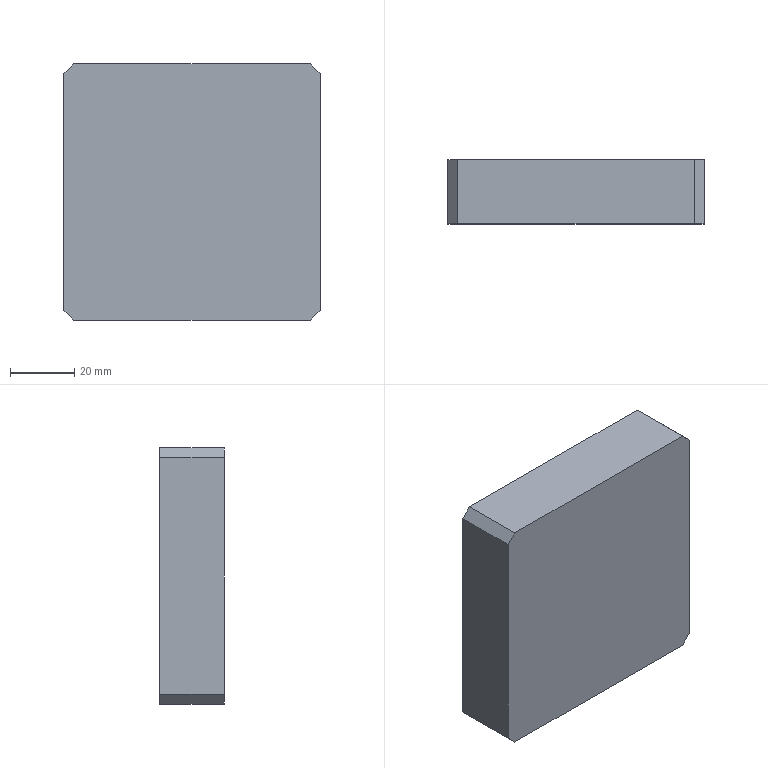Component | SolidWorks | CoilCarrier-10 | 1 solid | 24 faces | box 80 x 20 x 80 mm | volume 111580 mm3 | plane 24 | material Plain Carbon Steel
build123d program:
from build123d import *

# Parameters (mm, degrees)
SKETCH1_W           = 80
SKETCH1_H           = 80
BOSS_EXTRUDE1_DEPTH = 20
CUT_EXTRUDE1_DEPTH  = 11
CHAMFER1_SIZE       = 3
SKETCH3_W           = 14
SKETCH3_H           = 22
CUT_EXTRUDE2_DEPTH  = 1.25


with BuildPart() as part:
    # Sketch1 → Boss-Extrude1 (new body)
    with BuildSketch(Plane.XY):
        Rectangle(SKETCH1_W, SKETCH1_H)
    extrude(amount=BOSS_EXTRUDE1_DEPTH)

    # Sketch2 → Cut-Extrude1 (cut)
    with BuildSketch(Plane.XY.offset(20)):
        Polygon((12.5, -6), (12.5, -18), (-19.5, -18), (-19.5, -23), (-27.5, -23), (-27.5, -18), (-32.5, -18), (-32.5, -6), (-20, -6), (-20, 20), (-10.75, 20), (3.25, 20), (12.5, 20), align=None)
    extrude(amount=-CUT_EXTRUDE1_DEPTH, mode=Mode.SUBTRACT)

    # Chamfer1
    chamfer1_edges = [part.edges().sort_by_distance(p)[0] for p in [
        (-40, 40, 10),
        (40, 40, 10),
        (40, -40, 10),
        (-40, -40, 10),
    ]]
    chamfer(chamfer1_edges, length=CHAMFER1_SIZE)

    # Sketch3 → Cut-Extrude2 (cut)
    with BuildSketch(Plane.XY.offset(20)):
        with Locations((-3.75, -29)):
            Rectangle(SKETCH3_W, SKETCH3_H)
    extrude(amount=-CUT_EXTRUDE2_DEPTH, mode=Mode.SUBTRACT)


solid = part.part

# Placed as in the assembly
solid = solid.moved(Location((-4.55, 27.146, 668.775), (-90, 0, 90)))
STEP:
#1=COLOUR_RGB('',0.7922,0.8196,0.9333);
#2=FILL_AREA_STYLE_COLOUR('',#1);
#3=FILL_AREA_STYLE('',(#2));
#4=SURFACE_STYLE_FILL_AREA(#3);
#5=SURFACE_SIDE_STYLE('',(#4));
#6=SURFACE_STYLE_USAGE(.BOTH.,#5);
#7=PRESENTATION_STYLE_ASSIGNMENT((#6));
#8=CARTESIAN_POINT('',(-1.636,1.856,27.905));
#9=VERTEX_POINT('',#8);
#10=CARTESIAN_POINT('',(1.278,1.856,27.905));
#11=VERTEX_POINT('',#10);
#12=CARTESIAN_POINT('',(1.396,1.856,27.905));
#13=DIRECTION('',(1.,0.,0.));
#14=VECTOR('',#13,39.37);
#15=LINE('',#12,#14);
#16=EDGE_CURVE('',#9,#11,#15,.T.);
#17=ORIENTED_EDGE('',*,*,#16,.F.);
#18=CARTESIAN_POINT('',(-1.636,1.069,27.905));
#19=VERTEX_POINT('',#18);
#20=CARTESIAN_POINT('',(-1.636,1.856,27.905));
#21=DIRECTION('',(0.,-1.,-0.));
#22=VECTOR('',#21,39.37);
#23=LINE('',#20,#22);
#24=EDGE_CURVE('',#9,#19,#23,.T.);
#25=ORIENTED_EDGE('',*,*,#24,.T.);
#26=CARTESIAN_POINT('',(1.278,1.069,27.905));
#27=VERTEX_POINT('',#26);
#28=CARTESIAN_POINT('',(1.396,1.069,27.905));
#29=DIRECTION('',(1.,0.,0.));
#30=VECTOR('',#29,39.37);
#31=LINE('',#28,#30);
#32=EDGE_CURVE('',#19,#27,#31,.T.);
#33=ORIENTED_EDGE('',*,*,#32,.T.);
#34=CARTESIAN_POINT('',(1.278,1.856,27.905));
#35=DIRECTION('',(-0.,1.,0.));
#36=VECTOR('',#35,39.37);
#37=LINE('',#34,#36);
#38=EDGE_CURVE('',#27,#11,#37,.T.);
#39=ORIENTED_EDGE('',*,*,#38,.T.);
#40=EDGE_LOOP('',(#17,#25,#33,#39));
#41=FACE_OUTER_BOUND('',#40,.T.);
#42=CARTESIAN_POINT('',(1.396,1.856,27.905));
#43=DIRECTION('',(0.,0.,-1.));
#44=DIRECTION('',(0.,-1.,-0.));
#45=AXIS2_PLACEMENT_3D('',#42,#43,#44);
#46=PLANE('',#45);
#47=ADVANCED_FACE('',(#41),#46,.F.);
#48=CARTESIAN_POINT('',(1.396,1.807,26.753));
#49=VERTEX_POINT('',#48);
#50=CARTESIAN_POINT('',(1.396,1.807,26.202));
#51=VERTEX_POINT('',#50);
#52=CARTESIAN_POINT('',(1.396,1.807,26.753));
#53=DIRECTION('',(0.,0.,-1.));
#54=VECTOR('',#53,39.37);
#55=LINE('',#52,#54);
#56=EDGE_CURVE('',#49,#51,#55,.T.);
#57=ORIENTED_EDGE('',*,*,#56,.F.);
#58=CARTESIAN_POINT('',(1.396,1.856,26.753));
#59=VERTEX_POINT('',#58);
#60=CARTESIAN_POINT('',(1.396,1.807,26.753));
#61=DIRECTION('',(-0.,1.,0.));
#62=VECTOR('',#61,39.37);
#63=LINE('',#60,#62);
#64=EDGE_CURVE('',#49,#59,#63,.T.);
#65=ORIENTED_EDGE('',*,*,#64,.T.);
#66=CARTESIAN_POINT('',(1.396,1.856,27.786));
#67=VERTEX_POINT('',#66);
#68=CARTESIAN_POINT('',(1.396,1.856,24.755));
#69=DIRECTION('',(0.,0.,-1.));
#70=VECTOR('',#69,39.37);
#71=LINE('',#68,#70);
#72=EDGE_CURVE('',#67,#59,#71,.T.);
#73=ORIENTED_EDGE('',*,*,#72,.F.);
#74=CARTESIAN_POINT('',(1.396,1.069,27.786));
#75=VERTEX_POINT('',#74);
#76=CARTESIAN_POINT('',(1.396,1.856,27.786));
#77=DIRECTION('',(0.,-1.,-0.));
#78=VECTOR('',#77,39.37);
#79=LINE('',#76,#78);
#80=EDGE_CURVE('',#67,#75,#79,.T.);
#81=ORIENTED_EDGE('',*,*,#80,.T.);
#82=CARTESIAN_POINT('',(1.396,1.069,24.873));
#83=VERTEX_POINT('',#82);
#84=CARTESIAN_POINT('',(1.396,1.069,24.755));
#85=DIRECTION('',(0.,0.,-1.));
#86=VECTOR('',#85,39.37);
#87=LINE('',#84,#86);
#88=EDGE_CURVE('',#75,#83,#87,.T.);
#89=ORIENTED_EDGE('',*,*,#88,.T.);
#90=CARTESIAN_POINT('',(1.396,1.856,24.873));
#91=VERTEX_POINT('',#90);
#92=CARTESIAN_POINT('',(1.396,1.856,24.873));
#93=DIRECTION('',(-0.,1.,0.));
#94=VECTOR('',#93,39.37);
#95=LINE('',#92,#94);
#96=EDGE_CURVE('',#83,#91,#95,.T.);
#97=ORIENTED_EDGE('',*,*,#96,.T.);
#98=CARTESIAN_POINT('',(1.396,1.856,26.202));
#99=VERTEX_POINT('',#98);
#100=CARTESIAN_POINT('',(1.396,1.856,24.755));
#101=DIRECTION('',(0.,0.,-1.));
#102=VECTOR('',#101,39.37);
#103=LINE('',#100,#102);
#104=EDGE_CURVE('',#99,#91,#103,.T.);
#105=ORIENTED_EDGE('',*,*,#104,.F.);
#106=CARTESIAN_POINT('',(1.396,1.807,26.202));
#107=DIRECTION('',(-0.,1.,0.));
#108=VECTOR('',#107,39.37);
#109=LINE('',#106,#108);
#110=EDGE_CURVE('',#51,#99,#109,.T.);
#111=ORIENTED_EDGE('',*,*,#110,.F.);
#112=EDGE_LOOP('',(#57,#65,#73,#81,#89,#97,#105,#111));
#113=FACE_OUTER_BOUND('',#112,.T.);
#114=CARTESIAN_POINT('',(1.396,1.856,24.755));
#115=DIRECTION('',(-1.,-0.,-0.));
#116=DIRECTION('',(-0.,-0.,1.));
#117=AXIS2_PLACEMENT_3D('',#114,#115,#116);
#118=PLANE('',#117);
#119=ADVANCED_FACE('',(#113),#118,.F.);
#120=CARTESIAN_POINT('',(1.278,1.069,24.755));
#121=VERTEX_POINT('',#120);
#122=CARTESIAN_POINT('',(-1.636,1.069,24.755));
#123=VERTEX_POINT('',#122);
#124=CARTESIAN_POINT('',(1.396,1.069,24.755));
#125=DIRECTION('',(-1.,-0.,-0.));
#126=VECTOR('',#125,39.37);
#127=LINE('',#124,#126);
#128=EDGE_CURVE('',#121,#123,#127,.T.);
#129=ORIENTED_EDGE('',*,*,#128,.T.);
#130=CARTESIAN_POINT('',(-1.636,1.856,24.755));
#131=VERTEX_POINT('',#130);
#132=CARTESIAN_POINT('',(-1.636,1.856,24.755));
#133=DIRECTION('',(-0.,1.,0.));
#134=VECTOR('',#133,39.37);
#135=LINE('',#132,#134);
#136=EDGE_CURVE('',#123,#131,#135,.T.);
#137=ORIENTED_EDGE('',*,*,#136,.T.);
#138=CARTESIAN_POINT('',(1.278,1.856,24.755));
#139=VERTEX_POINT('',#138);
#140=CARTESIAN_POINT('',(1.396,1.856,24.755));
#141=DIRECTION('',(-1.,-0.,-0.));
#142=VECTOR('',#141,39.37);
#143=LINE('',#140,#142);
#144=EDGE_CURVE('',#139,#131,#143,.T.);
#145=ORIENTED_EDGE('',*,*,#144,.F.);
#146=CARTESIAN_POINT('',(1.278,1.856,24.755));
#147=DIRECTION('',(0.,-1.,-0.));
#148=VECTOR('',#147,39.37);
#149=LINE('',#146,#148);
#150=EDGE_CURVE('',#139,#121,#149,.T.);
#151=ORIENTED_EDGE('',*,*,#150,.T.);
#152=EDGE_LOOP('',(#129,#137,#145,#151));
#153=FACE_OUTER_BOUND('',#152,.T.);
#154=CARTESIAN_POINT('',(1.396,1.856,24.755));
#155=DIRECTION('',(-0.,-0.,1.));
#156=DIRECTION('',(-0.,1.,0.));
#157=AXIS2_PLACEMENT_3D('',#154,#155,#156);
#158=PLANE('',#157);
#159=ADVANCED_FACE('',(#153),#158,.F.);
#160=CARTESIAN_POINT('',(-1.754,1.856,24.873));
#161=VERTEX_POINT('',#160);
#162=CARTESIAN_POINT('',(-1.754,1.856,27.786));
#163=VERTEX_POINT('',#162);
#164=CARTESIAN_POINT('',(-1.754,1.856,24.755));
#165=DIRECTION('',(0.,-0.,1.));
#166=VECTOR('',#165,39.37);
#167=LINE('',#164,#166);
#168=EDGE_CURVE('',#161,#163,#167,.T.);
#169=ORIENTED_EDGE('',*,*,#168,.F.);
#170=CARTESIAN_POINT('',(-1.754,1.069,24.873));
#171=VERTEX_POINT('',#170);
#172=CARTESIAN_POINT('',(-1.754,1.856,24.873));
#173=DIRECTION('',(0.,-1.,-0.));
#174=VECTOR('',#173,39.37);
#175=LINE('',#172,#174);
#176=EDGE_CURVE('',#161,#171,#175,.T.);
#177=ORIENTED_EDGE('',*,*,#176,.T.);
#178=CARTESIAN_POINT('',(-1.754,1.069,27.786));
#179=VERTEX_POINT('',#178);
#180=CARTESIAN_POINT('',(-1.754,1.069,24.755));
#181=DIRECTION('',(0.,-0.,1.));
#182=VECTOR('',#181,39.37);
#183=LINE('',#180,#182);
#184=EDGE_CURVE('',#171,#179,#183,.T.);
#185=ORIENTED_EDGE('',*,*,#184,.T.);
#186=CARTESIAN_POINT('',(-1.754,1.856,27.786));
#187=DIRECTION('',(-0.,1.,0.));
#188=VECTOR('',#187,39.37);
#189=LINE('',#186,#188);
#190=EDGE_CURVE('',#179,#163,#189,.T.);
#191=ORIENTED_EDGE('',*,*,#190,.T.);
#192=EDGE_LOOP('',(#169,#177,#185,#191));
#193=FACE_OUTER_BOUND('',#192,.T.);
#194=CARTESIAN_POINT('',(-1.754,1.856,24.755));
#195=DIRECTION('',(1.,0.,-0.));
#196=DIRECTION('',(-0.,0.,-1.));
#197=AXIS2_PLACEMENT_3D('',#194,#195,#196);
#198=PLANE('',#197);
#199=ADVANCED_FACE('',(#193),#198,.F.);
#200=CARTESIAN_POINT('',(0.5295,1.856,26.753));
#201=VERTEX_POINT('',#200);
#202=CARTESIAN_POINT('',(0.5295,1.856,26.753));
#203=DIRECTION('',(1.,0.,0.));
#204=VECTOR('',#203,39.37);
#205=LINE('',#202,#204);
#206=EDGE_CURVE('',#201,#59,#205,.T.);
#207=ORIENTED_EDGE('',*,*,#206,.F.);
#208=CARTESIAN_POINT('',(0.5295,1.856,27.097));
#209=VERTEX_POINT('',#208);
#210=CARTESIAN_POINT('',(0.5295,1.856,25.838));
#211=DIRECTION('',(0.,0.,-1.));
#212=VECTOR('',#211,39.37);
#213=LINE('',#210,#212);
#214=EDGE_CURVE('',#209,#201,#213,.T.);
#215=ORIENTED_EDGE('',*,*,#214,.F.);
#216=CARTESIAN_POINT('',(0.7264,1.856,27.097));
#217=VERTEX_POINT('',#216);
#218=CARTESIAN_POINT('',(0.5295,1.856,27.097));
#219=DIRECTION('',(-1.,-0.,-0.));
#220=VECTOR('',#219,39.37);
#221=LINE('',#218,#220);
#222=EDGE_CURVE('',#217,#209,#221,.T.);
#223=ORIENTED_EDGE('',*,*,#222,.F.);
#224=CARTESIAN_POINT('',(0.7264,1.856,27.412));
#225=VERTEX_POINT('',#224);
#226=CARTESIAN_POINT('',(0.7264,1.856,27.412));
#227=DIRECTION('',(0.,0.,-1.));
#228=VECTOR('',#227,39.37);
#229=LINE('',#226,#228);
#230=EDGE_CURVE('',#225,#217,#229,.T.);
#231=ORIENTED_EDGE('',*,*,#230,.F.);
#232=CARTESIAN_POINT('',(0.5295,1.856,27.412));
#233=VERTEX_POINT('',#232);
#234=CARTESIAN_POINT('',(0.5295,1.856,27.412));
#235=DIRECTION('',(1.,0.,0.));
#236=VECTOR('',#235,39.37);
#237=LINE('',#234,#236);
#238=EDGE_CURVE('',#233,#225,#237,.T.);
#239=ORIENTED_EDGE('',*,*,#238,.F.);
#240=CARTESIAN_POINT('',(0.5295,1.856,27.609));
#241=VERTEX_POINT('',#240);
#242=CARTESIAN_POINT('',(0.5295,1.856,27.609));
#243=DIRECTION('',(0.,0.,-1.));
#244=VECTOR('',#243,39.37);
#245=LINE('',#242,#244);
#246=EDGE_CURVE('',#241,#233,#245,.T.);
#247=ORIENTED_EDGE('',*,*,#246,.F.);
#248=CARTESIAN_POINT('',(0.0571,1.856,27.609));
#249=VERTEX_POINT('',#248);
#250=CARTESIAN_POINT('',(0.0571,1.856,27.609));
#251=DIRECTION('',(1.,0.,0.));
#252=VECTOR('',#251,39.37);
#253=LINE('',#250,#252);
#254=EDGE_CURVE('',#249,#241,#253,.T.);
#255=ORIENTED_EDGE('',*,*,#254,.F.);
#256=CARTESIAN_POINT('',(0.0571,1.856,27.117));
#257=VERTEX_POINT('',#256);
#258=CARTESIAN_POINT('',(0.0571,1.856,27.117));
#259=DIRECTION('',(-0.,-0.,1.));
#260=VECTOR('',#259,39.37);
#261=LINE('',#258,#260);
#262=EDGE_CURVE('',#257,#249,#261,.T.);
#263=ORIENTED_EDGE('',*,*,#262,.F.);
#264=CARTESIAN_POINT('',(-0.9665,1.856,27.117));
#265=VERTEX_POINT('',#264);
#266=CARTESIAN_POINT('',(0.0571,1.856,27.117));
#267=DIRECTION('',(1.,0.,0.));
#268=VECTOR('',#267,39.37);
#269=LINE('',#266,#268);
#270=EDGE_CURVE('',#265,#257,#269,.T.);
#271=ORIENTED_EDGE('',*,*,#270,.F.);
#272=CARTESIAN_POINT('',(-0.9665,1.856,25.838));
#273=VERTEX_POINT('',#272);
#274=CARTESIAN_POINT('',(-0.9665,1.856,26.753));
#275=DIRECTION('',(-0.,-0.,1.));
#276=VECTOR('',#275,39.37);
#277=LINE('',#274,#276);
#278=EDGE_CURVE('',#273,#265,#277,.T.);
#279=ORIENTED_EDGE('',*,*,#278,.F.);
#280=CARTESIAN_POINT('',(0.5295,1.856,25.838));
#281=VERTEX_POINT('',#280);
#282=CARTESIAN_POINT('',(0.0571,1.856,25.838));
#283=DIRECTION('',(-1.,-0.,-0.));
#284=VECTOR('',#283,39.37);
#285=LINE('',#282,#284);
#286=EDGE_CURVE('',#281,#273,#285,.T.);
#287=ORIENTED_EDGE('',*,*,#286,.F.);
#288=CARTESIAN_POINT('',(0.5295,1.856,26.202));
#289=VERTEX_POINT('',#288);
#290=CARTESIAN_POINT('',(0.5295,1.856,25.838));
#291=DIRECTION('',(0.,0.,-1.));
#292=VECTOR('',#291,39.37);
#293=LINE('',#290,#292);
#294=EDGE_CURVE('',#289,#281,#293,.T.);
#295=ORIENTED_EDGE('',*,*,#294,.F.);
#296=CARTESIAN_POINT('',(0.5295,1.856,26.202));
#297=DIRECTION('',(-1.,-0.,0.));
#298=VECTOR('',#297,39.37);
#299=LINE('',#296,#298);
#300=EDGE_CURVE('',#99,#289,#299,.T.);
#301=ORIENTED_EDGE('',*,*,#300,.F.);
#302=ORIENTED_EDGE('',*,*,#104,.T.);
#303=CARTESIAN_POINT('',(1.337,1.856,24.814));
#304=DIRECTION('',(-0.7071,-0.,-0.7071));
#305=VECTOR('',#304,39.37);
#306=LINE('',#303,#305);
#307=EDGE_CURVE('',#91,#139,#306,.T.);
#308=ORIENTED_EDGE('',*,*,#307,.T.);
#309=ORIENTED_EDGE('',*,*,#144,.T.);
#310=CARTESIAN_POINT('',(-1.695,1.856,24.814));
#311=DIRECTION('',(-0.7071,-0.,0.7071));
#312=VECTOR('',#311,39.37);
#313=LINE('',#310,#312);
#314=EDGE_CURVE('',#131,#161,#313,.T.);
#315=ORIENTED_EDGE('',*,*,#314,.T.);
#316=ORIENTED_EDGE('',*,*,#168,.T.);
#317=CARTESIAN_POINT('',(-1.695,1.856,27.845));
#318=DIRECTION('',(0.7071,0.,0.7071));
#319=VECTOR('',#318,39.37);
#320=LINE('',#317,#319);
#321=EDGE_CURVE('',#163,#9,#320,.T.);
#322=ORIENTED_EDGE('',*,*,#321,.T.);
#323=ORIENTED_EDGE('',*,*,#16,.T.);
#324=CARTESIAN_POINT('',(1.337,1.856,27.845));
#325=DIRECTION('',(0.7071,0.,-0.7071));
#326=VECTOR('',#325,39.37);
#327=LINE('',#324,#326);
#328=EDGE_CURVE('',#11,#67,#327,.T.);
#329=ORIENTED_EDGE('',*,*,#328,.T.);
#330=ORIENTED_EDGE('',*,*,#72,.T.);
#331=EDGE_LOOP('',(#207,#215,#223,#231,#239,#247,#255,#263,#271,#279,#287,#295,#301,#302,#308,#309,#315,#316,#322,#323,#329,#330));
#332=FACE_OUTER_BOUND('',#331,.T.);
#333=CARTESIAN_POINT('',(-0.1791,1.856,26.33));
#334=DIRECTION('',(-0.,1.,0.));
#335=DIRECTION('',(0.,0.,-1.));
#336=AXIS2_PLACEMENT_3D('',#333,#334,#335);
#337=PLANE('',#336);
#338=ADVANCED_FACE('',(#332),#337,.T.);
#339=ORIENTED_EDGE('',*,*,#184,.F.);
#340=CARTESIAN_POINT('',(-1.754,1.069,24.873));
#341=DIRECTION('',(0.7071,0.,-0.7071));
#342=VECTOR('',#341,39.37);
#343=LINE('',#340,#342);
#344=EDGE_CURVE('',#171,#123,#343,.T.);
#345=ORIENTED_EDGE('',*,*,#344,.T.);
#346=ORIENTED_EDGE('',*,*,#128,.F.);
#347=CARTESIAN_POINT('',(1.278,1.069,24.755));
#348=DIRECTION('',(0.7071,0.,0.7071));
#349=VECTOR('',#348,39.37);
#350=LINE('',#347,#349);
#351=EDGE_CURVE('',#121,#83,#350,.T.);
#352=ORIENTED_EDGE('',*,*,#351,.T.);
#353=ORIENTED_EDGE('',*,*,#88,.F.);
#354=CARTESIAN_POINT('',(1.396,1.069,27.786));
#355=DIRECTION('',(-0.7071,-0.,0.7071));
#356=VECTOR('',#355,39.37);
#357=LINE('',#354,#356);
#358=EDGE_CURVE('',#75,#27,#357,.T.);
#359=ORIENTED_EDGE('',*,*,#358,.T.);
#360=ORIENTED_EDGE('',*,*,#32,.F.);
#361=CARTESIAN_POINT('',(-1.636,1.069,27.905));
#362=DIRECTION('',(-0.7071,-0.,-0.7071));
#363=VECTOR('',#362,39.37);
#364=LINE('',#361,#363);
#365=EDGE_CURVE('',#19,#179,#364,.T.);
#366=ORIENTED_EDGE('',*,*,#365,.T.);
#367=EDGE_LOOP('',(#339,#345,#346,#352,#353,#359,#360,#366));
#368=FACE_OUTER_BOUND('',#367,.T.);
#369=CARTESIAN_POINT('',(-0.1791,1.069,26.33));
#370=DIRECTION('',(-0.,1.,0.));
#371=DIRECTION('',(0.,0.,-1.));
#372=AXIS2_PLACEMENT_3D('',#369,#370,#371);
#373=PLANE('',#372);
#374=ADVANCED_FACE('',(#368),#373,.F.);
#375=ORIENTED_EDGE('',*,*,#278,.T.);
#376=CARTESIAN_POINT('',(-0.9665,1.423,27.117));
#377=VERTEX_POINT('',#376);
#378=CARTESIAN_POINT('',(-0.9665,1.423,27.117));
#379=DIRECTION('',(-0.,1.,0.));
#380=VECTOR('',#379,39.37);
#381=LINE('',#378,#380);
#382=EDGE_CURVE('',#377,#265,#381,.T.);
#383=ORIENTED_EDGE('',*,*,#382,.F.);
#384=CARTESIAN_POINT('',(-0.9665,1.423,25.838));
#385=VERTEX_POINT('',#384);
#386=CARTESIAN_POINT('',(-0.9665,1.423,26.753));
#387=DIRECTION('',(0.,-0.,1.));
#388=VECTOR('',#387,39.37);
#389=LINE('',#386,#388);
#390=EDGE_CURVE('',#385,#377,#389,.T.);
#391=ORIENTED_EDGE('',*,*,#390,.F.);
#392=CARTESIAN_POINT('',(-0.9665,1.423,25.838));
#393=DIRECTION('',(-0.,1.,0.));
#394=VECTOR('',#393,39.37);
#395=LINE('',#392,#394);
#396=EDGE_CURVE('',#385,#273,#395,.T.);
#397=ORIENTED_EDGE('',*,*,#396,.T.);
#398=EDGE_LOOP('',(#375,#383,#391,#397));
#399=FACE_OUTER_BOUND('',#398,.T.);
#400=CARTESIAN_POINT('',(-0.9665,1.423,26.753));
#401=DIRECTION('',(-1.,-0.,-0.));
#402=DIRECTION('',(-0.,1.,0.));
#403=AXIS2_PLACEMENT_3D('',#400,#401,#402);
#404=PLANE('',#403);
#405=ADVANCED_FACE('',(#399),#404,.F.);
#406=ORIENTED_EDGE('',*,*,#286,.T.);
#407=ORIENTED_EDGE('',*,*,#396,.F.);
#408=CARTESIAN_POINT('',(0.5295,1.423,25.838));
#409=VERTEX_POINT('',#408);
#410=CARTESIAN_POINT('',(0.0571,1.423,25.838));
#411=DIRECTION('',(-1.,-0.,-0.));
#412=VECTOR('',#411,39.37);
#413=LINE('',#410,#412);
#414=EDGE_CURVE('',#409,#385,#413,.T.);
#415=ORIENTED_EDGE('',*,*,#414,.F.);
#416=CARTESIAN_POINT('',(0.5295,1.423,25.838));
#417=DIRECTION('',(-0.,1.,0.));
#418=VECTOR('',#417,39.37);
#419=LINE('',#416,#418);
#420=EDGE_CURVE('',#409,#281,#419,.T.);
#421=ORIENTED_EDGE('',*,*,#420,.T.);
#422=EDGE_LOOP('',(#406,#407,#415,#421));
#423=FACE_OUTER_BOUND('',#422,.T.);
#424=CARTESIAN_POINT('',(0.0571,1.423,25.838));
#425=DIRECTION('',(0.,0.,-1.));
#426=DIRECTION('',(0.,-1.,-0.));
#427=AXIS2_PLACEMENT_3D('',#424,#425,#426);
#428=PLANE('',#427);
#429=ADVANCED_FACE('',(#423),#428,.F.);
#430=ORIENTED_EDGE('',*,*,#214,.T.);
#431=CARTESIAN_POINT('',(0.5295,1.807,26.753));
#432=VERTEX_POINT('',#431);
#433=CARTESIAN_POINT('',(0.5295,1.807,26.753));
#434=DIRECTION('',(-0.,1.,0.));
#435=VECTOR('',#434,39.37);
#436=LINE('',#433,#435);
#437=EDGE_CURVE('',#432,#201,#436,.T.);
#438=ORIENTED_EDGE('',*,*,#437,.F.);
#439=CARTESIAN_POINT('',(0.5295,1.807,26.202));
#440=VERTEX_POINT('',#439);
#441=CARTESIAN_POINT('',(0.5295,1.807,26.753));
#442=DIRECTION('',(-0.,-0.,1.));
#443=VECTOR('',#442,39.37);
#444=LINE('',#441,#443);
#445=EDGE_CURVE('',#440,#432,#444,.T.);
#446=ORIENTED_EDGE('',*,*,#445,.F.);
#447=CARTESIAN_POINT('',(0.5295,1.807,26.202));
#448=DIRECTION('',(-0.,1.,0.));
#449=VECTOR('',#448,39.37);
#450=LINE('',#447,#449);
#451=EDGE_CURVE('',#440,#289,#450,.T.);
#452=ORIENTED_EDGE('',*,*,#451,.T.);
#453=ORIENTED_EDGE('',*,*,#294,.T.);
#454=ORIENTED_EDGE('',*,*,#420,.F.);
#455=CARTESIAN_POINT('',(0.5295,1.423,27.097));
#456=VERTEX_POINT('',#455);
#457=CARTESIAN_POINT('',(0.5295,1.423,25.838));
#458=DIRECTION('',(0.,0.,-1.));
#459=VECTOR('',#458,39.37);
#460=LINE('',#457,#459);
#461=EDGE_CURVE('',#456,#409,#460,.T.);
#462=ORIENTED_EDGE('',*,*,#461,.F.);
#463=CARTESIAN_POINT('',(0.5295,1.423,27.097));
#464=DIRECTION('',(-0.,1.,0.));
#465=VECTOR('',#464,39.37);
#466=LINE('',#463,#465);
#467=EDGE_CURVE('',#456,#209,#466,.T.);
#468=ORIENTED_EDGE('',*,*,#467,.T.);
#469=EDGE_LOOP('',(#430,#438,#446,#452,#453,#454,#462,#468));
#470=FACE_OUTER_BOUND('',#469,.T.);
#471=CARTESIAN_POINT('',(0.5295,1.423,25.838));
#472=DIRECTION('',(1.,0.,0.));
#473=DIRECTION('',(0.,-1.,-0.));
#474=AXIS2_PLACEMENT_3D('',#471,#472,#473);
#475=PLANE('',#474);
#476=ADVANCED_FACE('',(#470),#475,.F.);
#477=ORIENTED_EDGE('',*,*,#222,.T.);
#478=ORIENTED_EDGE('',*,*,#467,.F.);
#479=CARTESIAN_POINT('',(0.7264,1.423,27.097));
#480=VERTEX_POINT('',#479);
#481=CARTESIAN_POINT('',(0.5295,1.423,27.097));
#482=DIRECTION('',(-1.,-0.,-0.));
#483=VECTOR('',#482,39.37);
#484=LINE('',#481,#483);
#485=EDGE_CURVE('',#480,#456,#484,.T.);
#486=ORIENTED_EDGE('',*,*,#485,.F.);
#487=CARTESIAN_POINT('',(0.7264,1.423,27.097));
#488=DIRECTION('',(-0.,1.,0.));
#489=VECTOR('',#488,39.37);
#490=LINE('',#487,#489);
#491=EDGE_CURVE('',#480,#217,#490,.T.);
#492=ORIENTED_EDGE('',*,*,#491,.T.);
#493=EDGE_LOOP('',(#477,#478,#486,#492));
#494=FACE_OUTER_BOUND('',#493,.T.);
#495=CARTESIAN_POINT('',(0.5295,1.423,27.097));
#496=DIRECTION('',(0.,0.,-1.));
#497=DIRECTION('',(0.,-1.,-0.));
#498=AXIS2_PLACEMENT_3D('',#495,#496,#497);
#499=PLANE('',#498);
#500=ADVANCED_FACE('',(#494),#499,.F.);
#501=ORIENTED_EDGE('',*,*,#230,.T.);
#502=ORIENTED_EDGE('',*,*,#491,.F.);
#503=CARTESIAN_POINT('',(0.7264,1.423,27.412));
#504=VERTEX_POINT('',#503);
#505=CARTESIAN_POINT('',(0.7264,1.423,27.412));
#506=DIRECTION('',(0.,0.,-1.));
#507=VECTOR('',#506,39.37);
#508=LINE('',#505,#507);
#509=EDGE_CURVE('',#504,#480,#508,.T.);
#510=ORIENTED_EDGE('',*,*,#509,.F.);
#511=CARTESIAN_POINT('',(0.7264,1.423,27.412));
#512=DIRECTION('',(-0.,1.,0.));
#513=VECTOR('',#512,39.37);
#514=LINE('',#511,#513);
#515=EDGE_CURVE('',#504,#225,#514,.T.);
#516=ORIENTED_EDGE('',*,*,#515,.T.);
#517=EDGE_LOOP('',(#501,#502,#510,#516));
#518=FACE_OUTER_BOUND('',#517,.T.);
#519=CARTESIAN_POINT('',(0.7264,1.423,27.412));
#520=DIRECTION('',(1.,0.,0.));
#521=DIRECTION('',(0.,-1.,-0.));
#522=AXIS2_PLACEMENT_3D('',#519,#520,#521);
#523=PLANE('',#522);
#524=ADVANCED_FACE('',(#518),#523,.F.);
#525=ORIENTED_EDGE('',*,*,#238,.T.);
#526=ORIENTED_EDGE('',*,*,#515,.F.);
#527=CARTESIAN_POINT('',(0.5295,1.423,27.412));
#528=VERTEX_POINT('',#527);
#529=CARTESIAN_POINT('',(0.5295,1.423,27.412));
#530=DIRECTION('',(1.,0.,0.));
#531=VECTOR('',#530,39.37);
#532=LINE('',#529,#531);
#533=EDGE_CURVE('',#528,#504,#532,.T.);
#534=ORIENTED_EDGE('',*,*,#533,.F.);
#535=CARTESIAN_POINT('',(0.5295,1.423,27.412));
#536=DIRECTION('',(-0.,1.,0.));
#537=VECTOR('',#536,39.37);
#538=LINE('',#535,#537);
#539=EDGE_CURVE('',#528,#233,#538,.T.);
#540=ORIENTED_EDGE('',*,*,#539,.T.);
#541=EDGE_LOOP('',(#525,#526,#534,#540));
#542=FACE_OUTER_BOUND('',#541,.T.);
#543=CARTESIAN_POINT('',(0.5295,1.423,27.412));
#544=DIRECTION('',(-0.,-0.,1.));
#545=DIRECTION('',(-0.,1.,0.));
#546=AXIS2_PLACEMENT_3D('',#543,#544,#545);
#547=PLANE('',#546);
#548=ADVANCED_FACE('',(#542),#547,.F.);
#549=ORIENTED_EDGE('',*,*,#246,.T.);
#550=ORIENTED_EDGE('',*,*,#539,.F.);
#551=CARTESIAN_POINT('',(0.5295,1.423,27.609));
#552=VERTEX_POINT('',#551);
#553=CARTESIAN_POINT('',(0.5295,1.423,27.609));
#554=DIRECTION('',(0.,0.,-1.));
#555=VECTOR('',#554,39.37);
#556=LINE('',#553,#555);
#557=EDGE_CURVE('',#552,#528,#556,.T.);
#558=ORIENTED_EDGE('',*,*,#557,.F.);
#559=CARTESIAN_POINT('',(0.5295,1.423,27.609));
#560=DIRECTION('',(-0.,1.,0.));
#561=VECTOR('',#560,39.37);
#562=LINE('',#559,#561);
#563=EDGE_CURVE('',#552,#241,#562,.T.);
#564=ORIENTED_EDGE('',*,*,#563,.T.);
#565=EDGE_LOOP('',(#549,#550,#558,#564));
#566=FACE_OUTER_BOUND('',#565,.T.);
#567=CARTESIAN_POINT('',(0.5295,1.423,27.609));
#568=DIRECTION('',(1.,0.,0.));
#569=DIRECTION('',(0.,-1.,-0.));
#570=AXIS2_PLACEMENT_3D('',#567,#568,#569);
#571=PLANE('',#570);
#572=ADVANCED_FACE('',(#566),#571,.F.);
#573=ORIENTED_EDGE('',*,*,#254,.T.);
#574=ORIENTED_EDGE('',*,*,#563,.F.);
#575=CARTESIAN_POINT('',(0.0571,1.423,27.609));
#576=VERTEX_POINT('',#575);
#577=CARTESIAN_POINT('',(0.0571,1.423,27.609));
#578=DIRECTION('',(1.,0.,0.));
#579=VECTOR('',#578,39.37);
#580=LINE('',#577,#579);
#581=EDGE_CURVE('',#576,#552,#580,.T.);
#582=ORIENTED_EDGE('',*,*,#581,.F.);
#583=CARTESIAN_POINT('',(0.0571,1.423,27.609));
#584=DIRECTION('',(-0.,1.,0.));
#585=VECTOR('',#584,39.37);
#586=LINE('',#583,#585);
#587=EDGE_CURVE('',#576,#249,#586,.T.);
#588=ORIENTED_EDGE('',*,*,#587,.T.);
#589=EDGE_LOOP('',(#573,#574,#582,#588));
#590=FACE_OUTER_BOUND('',#589,.T.);
#591=CARTESIAN_POINT('',(0.0571,1.423,27.609));
#592=DIRECTION('',(-0.,-0.,1.));
#593=DIRECTION('',(-0.,1.,0.));
#594=AXIS2_PLACEMENT_3D('',#591,#592,#593);
#595=PLANE('',#594);
#596=ADVANCED_FACE('',(#590),#595,.F.);
#597=ORIENTED_EDGE('',*,*,#262,.T.);
#598=ORIENTED_EDGE('',*,*,#587,.F.);
#599=CARTESIAN_POINT('',(0.0571,1.423,27.117));
#600=VERTEX_POINT('',#599);
#601=CARTESIAN_POINT('',(0.0571,1.423,27.117));
#602=DIRECTION('',(-0.,-0.,1.));
#603=VECTOR('',#602,39.37);
#604=LINE('',#601,#603);
#605=EDGE_CURVE('',#600,#576,#604,.T.);
#606=ORIENTED_EDGE('',*,*,#605,.F.);
#607=CARTESIAN_POINT('',(0.0571,1.423,27.117));
#608=DIRECTION('',(-0.,1.,0.));
#609=VECTOR('',#608,39.37);
#610=LINE('',#607,#609);
#611=EDGE_CURVE('',#600,#257,#610,.T.);
#612=ORIENTED_EDGE('',*,*,#611,.T.);
#613=EDGE_LOOP('',(#597,#598,#606,#612));
#614=FACE_OUTER_BOUND('',#613,.T.);
#615=CARTESIAN_POINT('',(0.0571,1.423,27.117));
#616=DIRECTION('',(-1.,-0.,-0.));
#617=DIRECTION('',(-0.,1.,0.));
#618=AXIS2_PLACEMENT_3D('',#615,#616,#617);
#619=PLANE('',#618);
#620=ADVANCED_FACE('',(#614),#619,.F.);
#621=ORIENTED_EDGE('',*,*,#270,.T.);
#622=ORIENTED_EDGE('',*,*,#611,.F.);
#623=CARTESIAN_POINT('',(0.0571,1.423,27.117));
#624=DIRECTION('',(1.,0.,0.));
#625=VECTOR('',#624,39.37);
#626=LINE('',#623,#625);
#627=EDGE_CURVE('',#377,#600,#626,.T.);
#628=ORIENTED_EDGE('',*,*,#627,.F.);
#629=ORIENTED_EDGE('',*,*,#382,.T.);
#630=EDGE_LOOP('',(#621,#622,#628,#629));
#631=FACE_OUTER_BOUND('',#630,.T.);
#632=CARTESIAN_POINT('',(0.0571,1.423,27.117));
#633=DIRECTION('',(-0.,-0.,1.));
#634=DIRECTION('',(-0.,1.,0.));
#635=AXIS2_PLACEMENT_3D('',#632,#633,#634);
#636=PLANE('',#635);
#637=ADVANCED_FACE('',(#631),#636,.F.);
#638=ORIENTED_EDGE('',*,*,#390,.T.);
#639=ORIENTED_EDGE('',*,*,#627,.T.);
#640=ORIENTED_EDGE('',*,*,#605,.T.);
#641=ORIENTED_EDGE('',*,*,#581,.T.);
#642=ORIENTED_EDGE('',*,*,#557,.T.);
#643=ORIENTED_EDGE('',*,*,#533,.T.);
#644=ORIENTED_EDGE('',*,*,#509,.T.);
#645=ORIENTED_EDGE('',*,*,#485,.T.);
#646=ORIENTED_EDGE('',*,*,#461,.T.);
#647=ORIENTED_EDGE('',*,*,#414,.T.);
#648=EDGE_LOOP('',(#638,#639,#640,#641,#642,#643,#644,#645,#646,#647));
#649=FACE_OUTER_BOUND('',#648,.T.);
#650=CARTESIAN_POINT('',(-0.1791,1.423,26.33));
#651=DIRECTION('',(0.,-1.,-0.));
#652=DIRECTION('',(-0.,-0.,1.));
#653=AXIS2_PLACEMENT_3D('',#650,#651,#652);
#654=PLANE('',#653);
#655=ADVANCED_FACE('',(#649),#654,.F.);
#656=ORIENTED_EDGE('',*,*,#314,.F.);
#657=ORIENTED_EDGE('',*,*,#136,.F.);
#658=ORIENTED_EDGE('',*,*,#344,.F.);
#659=ORIENTED_EDGE('',*,*,#176,.F.);
#660=EDGE_LOOP('',(#656,#657,#658,#659));
#661=FACE_OUTER_BOUND('',#660,.T.);
#662=CARTESIAN_POINT('',(-1.754,1.856,24.873));
#663=DIRECTION('',(0.7071,0.,0.7071));
#664=DIRECTION('',(0.,-1.,-0.));
#665=AXIS2_PLACEMENT_3D('',#662,#663,#664);
#666=PLANE('',#665);
#667=ADVANCED_FACE('',(#661),#666,.F.);
#668=ORIENTED_EDGE('',*,*,#321,.F.);
#669=ORIENTED_EDGE('',*,*,#190,.F.);
#670=ORIENTED_EDGE('',*,*,#365,.F.);
#671=ORIENTED_EDGE('',*,*,#24,.F.);
#672=EDGE_LOOP('',(#668,#669,#670,#671));
#673=FACE_OUTER_BOUND('',#672,.T.);
#674=CARTESIAN_POINT('',(-1.636,1.856,27.905));
#675=DIRECTION('',(0.7071,0.,-0.7071));
#676=DIRECTION('',(0.,-1.,-0.));
#677=AXIS2_PLACEMENT_3D('',#674,#675,#676);
#678=PLANE('',#677);
#679=ADVANCED_FACE('',(#673),#678,.F.);
#680=ORIENTED_EDGE('',*,*,#328,.F.);
#681=ORIENTED_EDGE('',*,*,#38,.F.);
#682=ORIENTED_EDGE('',*,*,#358,.F.);
#683=ORIENTED_EDGE('',*,*,#80,.F.);
#684=EDGE_LOOP('',(#680,#681,#682,#683));
#685=FACE_OUTER_BOUND('',#684,.T.);
#686=CARTESIAN_POINT('',(1.396,1.856,27.786));
#687=DIRECTION('',(-0.7071,-0.,-0.7071));
#688=DIRECTION('',(0.,-1.,-0.));
#689=AXIS2_PLACEMENT_3D('',#686,#687,#688);
#690=PLANE('',#689);
#691=ADVANCED_FACE('',(#685),#690,.F.);
#692=ORIENTED_EDGE('',*,*,#307,.F.);
#693=ORIENTED_EDGE('',*,*,#96,.F.);
#694=ORIENTED_EDGE('',*,*,#351,.F.);
#695=ORIENTED_EDGE('',*,*,#150,.F.);
#696=EDGE_LOOP('',(#692,#693,#694,#695));
#697=FACE_OUTER_BOUND('',#696,.T.);
#698=CARTESIAN_POINT('',(1.278,1.856,24.755));
#699=DIRECTION('',(-0.7071,-0.,0.7071));
#700=DIRECTION('',(0.,-1.,-0.));
#701=AXIS2_PLACEMENT_3D('',#698,#699,#700);
#702=PLANE('',#701);
#703=ADVANCED_FACE('',(#697),#702,.F.);
#704=ORIENTED_EDGE('',*,*,#206,.T.);
#705=ORIENTED_EDGE('',*,*,#64,.F.);
#706=CARTESIAN_POINT('',(0.5295,1.807,26.753));
#707=DIRECTION('',(1.,0.,0.));
#708=VECTOR('',#707,39.37);
#709=LINE('',#706,#708);
#710=EDGE_CURVE('',#432,#49,#709,.T.);
#711=ORIENTED_EDGE('',*,*,#710,.F.);
#712=ORIENTED_EDGE('',*,*,#437,.T.);
#713=EDGE_LOOP('',(#704,#705,#711,#712));
#714=FACE_OUTER_BOUND('',#713,.T.);
#715=CARTESIAN_POINT('',(0.5295,1.807,26.753));
#716=DIRECTION('',(-0.,-0.,1.));
#717=DIRECTION('',(1.,0.,0.));
#718=AXIS2_PLACEMENT_3D('',#715,#716,#717);
#719=PLANE('',#718);
#720=ADVANCED_FACE('',(#714),#719,.F.);
#721=ORIENTED_EDGE('',*,*,#300,.T.);
#722=ORIENTED_EDGE('',*,*,#451,.F.);
#723=CARTESIAN_POINT('',(0.5295,1.807,26.202));
#724=DIRECTION('',(-1.,-0.,0.));
#725=VECTOR('',#724,39.37);
#726=LINE('',#723,#725);
#727=EDGE_CURVE('',#51,#440,#726,.T.);
#728=ORIENTED_EDGE('',*,*,#727,.F.);
#729=ORIENTED_EDGE('',*,*,#110,.T.);
#730=EDGE_LOOP('',(#721,#722,#728,#729));
#731=FACE_OUTER_BOUND('',#730,.T.);
#732=CARTESIAN_POINT('',(0.5295,1.807,26.202));
#733=DIRECTION('',(-0.,0.,-1.));
#734=DIRECTION('',(-1.,-0.,0.));
#735=AXIS2_PLACEMENT_3D('',#732,#733,#734);
#736=PLANE('',#735);
#737=ADVANCED_FACE('',(#731),#736,.F.);
#738=ORIENTED_EDGE('',*,*,#710,.T.);
#739=ORIENTED_EDGE('',*,*,#56,.T.);
#740=ORIENTED_EDGE('',*,*,#727,.T.);
#741=ORIENTED_EDGE('',*,*,#445,.T.);
#742=EDGE_LOOP('',(#738,#739,#740,#741));
#743=FACE_OUTER_BOUND('',#742,.T.);
#744=CARTESIAN_POINT('',(-0.1791,1.807,26.33));
#745=DIRECTION('',(-0.,1.,0.));
#746=DIRECTION('',(0.,0.,-1.));
#747=AXIS2_PLACEMENT_3D('',#744,#745,#746);
#748=PLANE('',#747);
#749=ADVANCED_FACE('',(#743),#748,.T.);
#750=CLOSED_SHELL('',(#47,#119,#159,#199,#338,#374,#405,#429,#476,#500,#524,#548,#572,#596,#620,#637,#655,#667,#679,#691,#703,#720,#737,#749));
#751=MANIFOLD_SOLID_BREP('',#750);
#752=STYLED_ITEM('',(#7),#751);
#753=PRESENTATION_LAYER_ASSIGNMENT('','',(#752));
#754=CARTESIAN_POINT('',(0.,0.,0.));
#755=DIRECTION('',(0.,0.,1.));
#756=DIRECTION('',(1.,0.,0.));
#757=AXIS2_PLACEMENT_3D('',#754,#755,#756);
#758=(LENGTH_UNIT()NAMED_UNIT(*)SI_UNIT($,.METRE.));
#759=LENGTH_MEASURE_WITH_UNIT(LENGTH_MEASURE(0.0254),#758);
#760=DIMENSIONAL_EXPONENTS(1.,0.,0.,0.,0.,0.,0.);
#761=(CONVERSION_BASED_UNIT('',#759)LENGTH_UNIT()NAMED_UNIT(#760));
#762=UNCERTAINTY_MEASURE_WITH_UNIT(LENGTH_MEASURE(0.00001),#761,'','');
#763=(NAMED_UNIT(*)PLANE_ANGLE_UNIT()SI_UNIT($,.RADIAN.));
#764=(NAMED_UNIT(*)SI_UNIT($,.STERADIAN.)SOLID_ANGLE_UNIT());
#765=(GEOMETRIC_REPRESENTATION_CONTEXT(3)GLOBAL_UNCERTAINTY_ASSIGNED_CONTEXT((#762))GLOBAL_UNIT_ASSIGNED_CONTEXT((#761,#763,#764))REPRESENTATION_CONTEXT('',''));
#766=ADVANCED_BREP_SHAPE_REPRESENTATION('',(#751,#757),#765);
#767=(LENGTH_UNIT()NAMED_UNIT(*)SI_UNIT($,.METRE.));
#768=LENGTH_MEASURE_WITH_UNIT(LENGTH_MEASURE(0.0254),#767);
#769=DIMENSIONAL_EXPONENTS(1.,0.,0.,0.,0.,0.,0.);
#770=(CONVERSION_BASED_UNIT('',#768)LENGTH_UNIT()NAMED_UNIT(#769));
#771=UNCERTAINTY_MEASURE_WITH_UNIT(LENGTH_MEASURE(0.00001),#770,'','');
#772=(NAMED_UNIT(*)PLANE_ANGLE_UNIT()SI_UNIT($,.RADIAN.));
#773=(NAMED_UNIT(*)SI_UNIT($,.STERADIAN.)SOLID_ANGLE_UNIT());
#774=(GEOMETRIC_REPRESENTATION_CONTEXT(3)GLOBAL_UNCERTAINTY_ASSIGNED_CONTEXT((#771))GLOBAL_UNIT_ASSIGNED_CONTEXT((#770,#772,#773))REPRESENTATION_CONTEXT('',''));
#775=MECHANICAL_DESIGN_GEOMETRIC_PRESENTATION_REPRESENTATION('',(#752),#774);